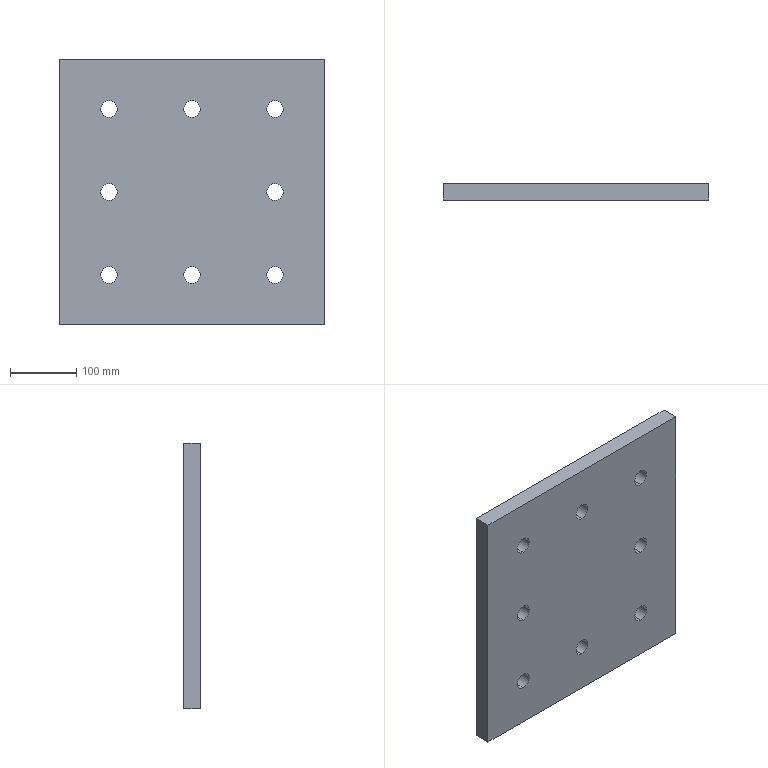Component | SolidWorks | SmallFlange25-2 | 1 solid | 22 faces | box 400 x 25 x 400 mm | volume 3901825 mm3 | cylinder 16 | plane 6 | commonest cylinder face diameters 25 x16 | material Plain Carbon Steel
STEP:
#1=COLOUR_RGB('',0.7922,0.8196,0.9333);
#2=FILL_AREA_STYLE_COLOUR('',#1);
#3=FILL_AREA_STYLE('',(#2));
#4=SURFACE_STYLE_FILL_AREA(#3);
#5=SURFACE_SIDE_STYLE('',(#4));
#6=SURFACE_STYLE_USAGE(.BOTH.,#5);
#7=PRESENTATION_STYLE_ASSIGNMENT((#6));
#8=CARTESIAN_POINT('',(21.257,113.181,151.881));
#9=VERTEX_POINT('',#8);
#10=CARTESIAN_POINT('',(21.257,113.181,152.866));
#11=VERTEX_POINT('',#10);
#12=CARTESIAN_POINT('',(21.257,113.181,152.374));
#13=DIRECTION('',(0.,1.,0.));
#14=DIRECTION('',(0.,0.,1.));
#15=AXIS2_PLACEMENT_3D('',#12,#13,#14);
#16=CIRCLE('',#15,0.4921);
#17=EDGE_CURVE('',#9,#11,#16,.T.);
#18=ORIENTED_EDGE('',*,*,#17,.F.);
#19=CARTESIAN_POINT('',(21.257,114.165,151.881));
#20=VERTEX_POINT('',#19);
#21=CARTESIAN_POINT('',(21.257,113.181,151.881));
#22=DIRECTION('',(0.,1.,0.));
#23=VECTOR('',#22,39.37);
#24=LINE('',#21,#23);
#25=EDGE_CURVE('',#9,#20,#24,.T.);
#26=ORIENTED_EDGE('',*,*,#25,.T.);
#27=CARTESIAN_POINT('',(21.257,114.165,152.866));
#28=VERTEX_POINT('',#27);
#29=CARTESIAN_POINT('',(21.257,114.165,152.374));
#30=DIRECTION('',(0.,1.,0.));
#31=DIRECTION('',(0.,0.,1.));
#32=AXIS2_PLACEMENT_3D('',#29,#30,#31);
#33=CIRCLE('',#32,0.4921);
#34=EDGE_CURVE('',#20,#28,#33,.T.);
#35=ORIENTED_EDGE('',*,*,#34,.T.);
#36=CARTESIAN_POINT('',(21.257,113.181,152.866));
#37=DIRECTION('',(0.,1.,0.));
#38=VECTOR('',#37,39.37);
#39=LINE('',#36,#38);
#40=EDGE_CURVE('',#11,#28,#39,.T.);
#41=ORIENTED_EDGE('',*,*,#40,.F.);
#42=EDGE_LOOP('',(#18,#26,#35,#41));
#43=FACE_OUTER_BOUND('',#42,.T.);
#44=CARTESIAN_POINT('',(21.257,113.181,152.374));
#45=DIRECTION('',(0.,1.,0.));
#46=DIRECTION('',(0.,0.,1.));
#47=AXIS2_PLACEMENT_3D('',#44,#45,#46);
#48=CYLINDRICAL_SURFACE('',#47,0.4921);
#49=ADVANCED_FACE('',(#43),#48,.F.);
#50=CARTESIAN_POINT('',(21.257,113.181,146.96));
#51=VERTEX_POINT('',#50);
#52=CARTESIAN_POINT('',(21.257,113.181,147.944));
#53=VERTEX_POINT('',#52);
#54=CARTESIAN_POINT('',(21.257,113.181,147.452));
#55=DIRECTION('',(0.,1.,0.));
#56=DIRECTION('',(0.,0.,1.));
#57=AXIS2_PLACEMENT_3D('',#54,#55,#56);
#58=CIRCLE('',#57,0.4921);
#59=EDGE_CURVE('',#51,#53,#58,.T.);
#60=ORIENTED_EDGE('',*,*,#59,.F.);
#61=CARTESIAN_POINT('',(21.257,114.165,146.96));
#62=VERTEX_POINT('',#61);
#63=CARTESIAN_POINT('',(21.257,113.181,146.96));
#64=DIRECTION('',(0.,1.,0.));
#65=VECTOR('',#64,39.37);
#66=LINE('',#63,#65);
#67=EDGE_CURVE('',#51,#62,#66,.T.);
#68=ORIENTED_EDGE('',*,*,#67,.T.);
#69=CARTESIAN_POINT('',(21.257,114.165,147.944));
#70=VERTEX_POINT('',#69);
#71=CARTESIAN_POINT('',(21.257,114.165,147.452));
#72=DIRECTION('',(0.,1.,0.));
#73=DIRECTION('',(0.,0.,1.));
#74=AXIS2_PLACEMENT_3D('',#71,#72,#73);
#75=CIRCLE('',#74,0.4921);
#76=EDGE_CURVE('',#62,#70,#75,.T.);
#77=ORIENTED_EDGE('',*,*,#76,.T.);
#78=CARTESIAN_POINT('',(21.257,113.181,147.944));
#79=DIRECTION('',(0.,1.,0.));
#80=VECTOR('',#79,39.37);
#81=LINE('',#78,#80);
#82=EDGE_CURVE('',#53,#70,#81,.T.);
#83=ORIENTED_EDGE('',*,*,#82,.F.);
#84=EDGE_LOOP('',(#60,#68,#77,#83));
#85=FACE_OUTER_BOUND('',#84,.T.);
#86=CARTESIAN_POINT('',(21.257,113.181,147.452));
#87=DIRECTION('',(0.,1.,0.));
#88=DIRECTION('',(0.,0.,1.));
#89=AXIS2_PLACEMENT_3D('',#86,#87,#88);
#90=CYLINDRICAL_SURFACE('',#89,0.4921);
#91=ADVANCED_FACE('',(#85),#90,.F.);
#92=CARTESIAN_POINT('',(31.1,113.181,151.881));
#93=VERTEX_POINT('',#92);
#94=CARTESIAN_POINT('',(31.1,113.181,152.866));
#95=VERTEX_POINT('',#94);
#96=CARTESIAN_POINT('',(31.1,113.181,152.374));
#97=DIRECTION('',(0.,1.,0.));
#98=DIRECTION('',(0.,0.,1.));
#99=AXIS2_PLACEMENT_3D('',#96,#97,#98);
#100=CIRCLE('',#99,0.4921);
#101=EDGE_CURVE('',#93,#95,#100,.T.);
#102=ORIENTED_EDGE('',*,*,#101,.F.);
#103=CARTESIAN_POINT('',(31.1,114.165,151.881));
#104=VERTEX_POINT('',#103);
#105=CARTESIAN_POINT('',(31.1,113.181,151.881));
#106=DIRECTION('',(0.,1.,0.));
#107=VECTOR('',#106,39.37);
#108=LINE('',#105,#107);
#109=EDGE_CURVE('',#93,#104,#108,.T.);
#110=ORIENTED_EDGE('',*,*,#109,.T.);
#111=CARTESIAN_POINT('',(31.1,114.165,152.866));
#112=VERTEX_POINT('',#111);
#113=CARTESIAN_POINT('',(31.1,114.165,152.374));
#114=DIRECTION('',(0.,1.,0.));
#115=DIRECTION('',(0.,0.,1.));
#116=AXIS2_PLACEMENT_3D('',#113,#114,#115);
#117=CIRCLE('',#116,0.4921);
#118=EDGE_CURVE('',#104,#112,#117,.T.);
#119=ORIENTED_EDGE('',*,*,#118,.T.);
#120=CARTESIAN_POINT('',(31.1,113.181,152.866));
#121=DIRECTION('',(0.,1.,0.));
#122=VECTOR('',#121,39.37);
#123=LINE('',#120,#122);
#124=EDGE_CURVE('',#95,#112,#123,.T.);
#125=ORIENTED_EDGE('',*,*,#124,.F.);
#126=EDGE_LOOP('',(#102,#110,#119,#125));
#127=FACE_OUTER_BOUND('',#126,.T.);
#128=CARTESIAN_POINT('',(31.1,113.181,152.374));
#129=DIRECTION('',(0.,1.,0.));
#130=DIRECTION('',(0.,0.,1.));
#131=AXIS2_PLACEMENT_3D('',#128,#129,#130);
#132=CYLINDRICAL_SURFACE('',#131,0.4921);
#133=ADVANCED_FACE('',(#127),#132,.F.);
#134=CARTESIAN_POINT('',(26.179,113.181,151.881));
#135=VERTEX_POINT('',#134);
#136=CARTESIAN_POINT('',(26.179,113.181,152.866));
#137=VERTEX_POINT('',#136);
#138=CARTESIAN_POINT('',(26.179,113.181,152.374));
#139=DIRECTION('',(0.,1.,0.));
#140=DIRECTION('',(0.,0.,1.));
#141=AXIS2_PLACEMENT_3D('',#138,#139,#140);
#142=CIRCLE('',#141,0.4921);
#143=EDGE_CURVE('',#135,#137,#142,.T.);
#144=ORIENTED_EDGE('',*,*,#143,.F.);
#145=CARTESIAN_POINT('',(26.179,114.165,151.881));
#146=VERTEX_POINT('',#145);
#147=CARTESIAN_POINT('',(26.179,113.181,151.881));
#148=DIRECTION('',(0.,1.,0.));
#149=VECTOR('',#148,39.37);
#150=LINE('',#147,#149);
#151=EDGE_CURVE('',#135,#146,#150,.T.);
#152=ORIENTED_EDGE('',*,*,#151,.T.);
#153=CARTESIAN_POINT('',(26.179,114.165,152.866));
#154=VERTEX_POINT('',#153);
#155=CARTESIAN_POINT('',(26.179,114.165,152.374));
#156=DIRECTION('',(0.,1.,0.));
#157=DIRECTION('',(0.,0.,1.));
#158=AXIS2_PLACEMENT_3D('',#155,#156,#157);
#159=CIRCLE('',#158,0.4921);
#160=EDGE_CURVE('',#146,#154,#159,.T.);
#161=ORIENTED_EDGE('',*,*,#160,.T.);
#162=CARTESIAN_POINT('',(26.179,113.181,152.866));
#163=DIRECTION('',(0.,1.,0.));
#164=VECTOR('',#163,39.37);
#165=LINE('',#162,#164);
#166=EDGE_CURVE('',#137,#154,#165,.T.);
#167=ORIENTED_EDGE('',*,*,#166,.F.);
#168=EDGE_LOOP('',(#144,#152,#161,#167));
#169=FACE_OUTER_BOUND('',#168,.T.);
#170=CARTESIAN_POINT('',(26.179,113.181,152.374));
#171=DIRECTION('',(0.,1.,0.));
#172=DIRECTION('',(0.,0.,1.));
#173=AXIS2_PLACEMENT_3D('',#170,#171,#172);
#174=CYLINDRICAL_SURFACE('',#173,0.4921);
#175=ADVANCED_FACE('',(#169),#174,.F.);
#176=CARTESIAN_POINT('',(31.1,113.181,146.96));
#177=VERTEX_POINT('',#176);
#178=CARTESIAN_POINT('',(31.1,113.181,147.944));
#179=VERTEX_POINT('',#178);
#180=CARTESIAN_POINT('',(31.1,113.181,147.452));
#181=DIRECTION('',(0.,1.,0.));
#182=DIRECTION('',(0.,0.,1.));
#183=AXIS2_PLACEMENT_3D('',#180,#181,#182);
#184=CIRCLE('',#183,0.4921);
#185=EDGE_CURVE('',#177,#179,#184,.T.);
#186=ORIENTED_EDGE('',*,*,#185,.F.);
#187=CARTESIAN_POINT('',(31.1,114.165,146.96));
#188=VERTEX_POINT('',#187);
#189=CARTESIAN_POINT('',(31.1,113.181,146.96));
#190=DIRECTION('',(0.,1.,0.));
#191=VECTOR('',#190,39.37);
#192=LINE('',#189,#191);
#193=EDGE_CURVE('',#177,#188,#192,.T.);
#194=ORIENTED_EDGE('',*,*,#193,.T.);
#195=CARTESIAN_POINT('',(31.1,114.165,147.944));
#196=VERTEX_POINT('',#195);
#197=CARTESIAN_POINT('',(31.1,114.165,147.452));
#198=DIRECTION('',(0.,1.,0.));
#199=DIRECTION('',(0.,0.,1.));
#200=AXIS2_PLACEMENT_3D('',#197,#198,#199);
#201=CIRCLE('',#200,0.4921);
#202=EDGE_CURVE('',#188,#196,#201,.T.);
#203=ORIENTED_EDGE('',*,*,#202,.T.);
#204=CARTESIAN_POINT('',(31.1,113.181,147.944));
#205=DIRECTION('',(0.,1.,0.));
#206=VECTOR('',#205,39.37);
#207=LINE('',#204,#206);
#208=EDGE_CURVE('',#179,#196,#207,.T.);
#209=ORIENTED_EDGE('',*,*,#208,.F.);
#210=EDGE_LOOP('',(#186,#194,#203,#209));
#211=FACE_OUTER_BOUND('',#210,.T.);
#212=CARTESIAN_POINT('',(31.1,113.181,147.452));
#213=DIRECTION('',(0.,1.,0.));
#214=DIRECTION('',(0.,0.,1.));
#215=AXIS2_PLACEMENT_3D('',#212,#213,#214);
#216=CYLINDRICAL_SURFACE('',#215,0.4921);
#217=ADVANCED_FACE('',(#211),#216,.F.);
#218=CARTESIAN_POINT('',(31.1,113.181,142.039));
#219=VERTEX_POINT('',#218);
#220=CARTESIAN_POINT('',(31.1,113.181,143.023));
#221=VERTEX_POINT('',#220);
#222=CARTESIAN_POINT('',(31.1,113.181,142.531));
#223=DIRECTION('',(0.,1.,0.));
#224=DIRECTION('',(0.,0.,1.));
#225=AXIS2_PLACEMENT_3D('',#222,#223,#224);
#226=CIRCLE('',#225,0.4921);
#227=EDGE_CURVE('',#219,#221,#226,.T.);
#228=ORIENTED_EDGE('',*,*,#227,.F.);
#229=CARTESIAN_POINT('',(31.1,114.165,142.039));
#230=VERTEX_POINT('',#229);
#231=CARTESIAN_POINT('',(31.1,113.181,142.039));
#232=DIRECTION('',(0.,1.,0.));
#233=VECTOR('',#232,39.37);
#234=LINE('',#231,#233);
#235=EDGE_CURVE('',#219,#230,#234,.T.);
#236=ORIENTED_EDGE('',*,*,#235,.T.);
#237=CARTESIAN_POINT('',(31.1,114.165,143.023));
#238=VERTEX_POINT('',#237);
#239=CARTESIAN_POINT('',(31.1,114.165,142.531));
#240=DIRECTION('',(0.,1.,0.));
#241=DIRECTION('',(0.,0.,1.));
#242=AXIS2_PLACEMENT_3D('',#239,#240,#241);
#243=CIRCLE('',#242,0.4921);
#244=EDGE_CURVE('',#230,#238,#243,.T.);
#245=ORIENTED_EDGE('',*,*,#244,.T.);
#246=CARTESIAN_POINT('',(31.1,113.181,143.023));
#247=DIRECTION('',(0.,1.,0.));
#248=VECTOR('',#247,39.37);
#249=LINE('',#246,#248);
#250=EDGE_CURVE('',#221,#238,#249,.T.);
#251=ORIENTED_EDGE('',*,*,#250,.F.);
#252=EDGE_LOOP('',(#228,#236,#245,#251));
#253=FACE_OUTER_BOUND('',#252,.T.);
#254=CARTESIAN_POINT('',(31.1,113.181,142.531));
#255=DIRECTION('',(0.,1.,0.));
#256=DIRECTION('',(0.,0.,1.));
#257=AXIS2_PLACEMENT_3D('',#254,#255,#256);
#258=CYLINDRICAL_SURFACE('',#257,0.4921);
#259=ADVANCED_FACE('',(#253),#258,.F.);
#260=CARTESIAN_POINT('',(26.179,113.181,142.039));
#261=VERTEX_POINT('',#260);
#262=CARTESIAN_POINT('',(26.179,113.181,143.023));
#263=VERTEX_POINT('',#262);
#264=CARTESIAN_POINT('',(26.179,113.181,142.531));
#265=DIRECTION('',(0.,1.,0.));
#266=DIRECTION('',(0.,0.,1.));
#267=AXIS2_PLACEMENT_3D('',#264,#265,#266);
#268=CIRCLE('',#267,0.4921);
#269=EDGE_CURVE('',#261,#263,#268,.T.);
#270=ORIENTED_EDGE('',*,*,#269,.F.);
#271=CARTESIAN_POINT('',(26.179,114.165,142.039));
#272=VERTEX_POINT('',#271);
#273=CARTESIAN_POINT('',(26.179,113.181,142.039));
#274=DIRECTION('',(0.,1.,0.));
#275=VECTOR('',#274,39.37);
#276=LINE('',#273,#275);
#277=EDGE_CURVE('',#261,#272,#276,.T.);
#278=ORIENTED_EDGE('',*,*,#277,.T.);
#279=CARTESIAN_POINT('',(26.179,114.165,143.023));
#280=VERTEX_POINT('',#279);
#281=CARTESIAN_POINT('',(26.179,114.165,142.531));
#282=DIRECTION('',(0.,1.,0.));
#283=DIRECTION('',(0.,0.,1.));
#284=AXIS2_PLACEMENT_3D('',#281,#282,#283);
#285=CIRCLE('',#284,0.4921);
#286=EDGE_CURVE('',#272,#280,#285,.T.);
#287=ORIENTED_EDGE('',*,*,#286,.T.);
#288=CARTESIAN_POINT('',(26.179,113.181,143.023));
#289=DIRECTION('',(0.,1.,0.));
#290=VECTOR('',#289,39.37);
#291=LINE('',#288,#290);
#292=EDGE_CURVE('',#263,#280,#291,.T.);
#293=ORIENTED_EDGE('',*,*,#292,.F.);
#294=EDGE_LOOP('',(#270,#278,#287,#293));
#295=FACE_OUTER_BOUND('',#294,.T.);
#296=CARTESIAN_POINT('',(26.179,113.181,142.531));
#297=DIRECTION('',(0.,1.,0.));
#298=DIRECTION('',(0.,0.,1.));
#299=AXIS2_PLACEMENT_3D('',#296,#297,#298);
#300=CYLINDRICAL_SURFACE('',#299,0.4921);
#301=ADVANCED_FACE('',(#295),#300,.F.);
#302=CARTESIAN_POINT('',(21.257,113.181,142.039));
#303=VERTEX_POINT('',#302);
#304=CARTESIAN_POINT('',(21.257,113.181,143.023));
#305=VERTEX_POINT('',#304);
#306=CARTESIAN_POINT('',(21.257,113.181,142.531));
#307=DIRECTION('',(0.,1.,0.));
#308=DIRECTION('',(0.,0.,1.));
#309=AXIS2_PLACEMENT_3D('',#306,#307,#308);
#310=CIRCLE('',#309,0.4921);
#311=EDGE_CURVE('',#303,#305,#310,.T.);
#312=ORIENTED_EDGE('',*,*,#311,.F.);
#313=CARTESIAN_POINT('',(21.257,114.165,142.039));
#314=VERTEX_POINT('',#313);
#315=CARTESIAN_POINT('',(21.257,113.181,142.039));
#316=DIRECTION('',(0.,1.,0.));
#317=VECTOR('',#316,39.37);
#318=LINE('',#315,#317);
#319=EDGE_CURVE('',#303,#314,#318,.T.);
#320=ORIENTED_EDGE('',*,*,#319,.T.);
#321=CARTESIAN_POINT('',(21.257,114.165,143.023));
#322=VERTEX_POINT('',#321);
#323=CARTESIAN_POINT('',(21.257,114.165,142.531));
#324=DIRECTION('',(0.,1.,0.));
#325=DIRECTION('',(0.,0.,1.));
#326=AXIS2_PLACEMENT_3D('',#323,#324,#325);
#327=CIRCLE('',#326,0.4921);
#328=EDGE_CURVE('',#314,#322,#327,.T.);
#329=ORIENTED_EDGE('',*,*,#328,.T.);
#330=CARTESIAN_POINT('',(21.257,113.181,143.023));
#331=DIRECTION('',(0.,1.,0.));
#332=VECTOR('',#331,39.37);
#333=LINE('',#330,#332);
#334=EDGE_CURVE('',#305,#322,#333,.T.);
#335=ORIENTED_EDGE('',*,*,#334,.F.);
#336=EDGE_LOOP('',(#312,#320,#329,#335));
#337=FACE_OUTER_BOUND('',#336,.T.);
#338=CARTESIAN_POINT('',(21.257,113.181,142.531));
#339=DIRECTION('',(0.,1.,0.));
#340=DIRECTION('',(0.,0.,1.));
#341=AXIS2_PLACEMENT_3D('',#338,#339,#340);
#342=CYLINDRICAL_SURFACE('',#341,0.4921);
#343=ADVANCED_FACE('',(#337),#342,.F.);
#344=CARTESIAN_POINT('',(34.053,114.165,155.326));
#345=VERTEX_POINT('',#344);
#346=CARTESIAN_POINT('',(34.053,114.165,139.578));
#347=VERTEX_POINT('',#346);
#348=CARTESIAN_POINT('',(34.053,114.165,139.578));
#349=DIRECTION('',(-0.,0.,-1.));
#350=VECTOR('',#349,39.37);
#351=LINE('',#348,#350);
#352=EDGE_CURVE('',#345,#347,#351,.T.);
#353=ORIENTED_EDGE('',*,*,#352,.F.);
#354=CARTESIAN_POINT('',(34.053,113.181,155.326));
#355=VERTEX_POINT('',#354);
#356=CARTESIAN_POINT('',(34.053,113.181,155.326));
#357=DIRECTION('',(0.,1.,0.));
#358=VECTOR('',#357,39.37);
#359=LINE('',#356,#358);
#360=EDGE_CURVE('',#355,#345,#359,.T.);
#361=ORIENTED_EDGE('',*,*,#360,.F.);
#362=CARTESIAN_POINT('',(34.053,113.181,139.578));
#363=VERTEX_POINT('',#362);
#364=CARTESIAN_POINT('',(34.053,113.181,139.578));
#365=DIRECTION('',(-0.,0.,-1.));
#366=VECTOR('',#365,39.37);
#367=LINE('',#364,#366);
#368=EDGE_CURVE('',#355,#363,#367,.T.);
#369=ORIENTED_EDGE('',*,*,#368,.T.);
#370=CARTESIAN_POINT('',(34.053,113.181,139.578));
#371=DIRECTION('',(0.,1.,0.));
#372=VECTOR('',#371,39.37);
#373=LINE('',#370,#372);
#374=EDGE_CURVE('',#363,#347,#373,.T.);
#375=ORIENTED_EDGE('',*,*,#374,.T.);
#376=EDGE_LOOP('',(#353,#361,#369,#375));
#377=FACE_OUTER_BOUND('',#376,.T.);
#378=CARTESIAN_POINT('',(34.053,113.181,139.578));
#379=DIRECTION('',(1.,0.,-0.));
#380=DIRECTION('',(-0.,0.,-1.));
#381=AXIS2_PLACEMENT_3D('',#378,#379,#380);
#382=PLANE('',#381);
#383=ADVANCED_FACE('',(#377),#382,.T.);
#384=CARTESIAN_POINT('',(18.305,114.165,155.326));
#385=VERTEX_POINT('',#384);
#386=CARTESIAN_POINT('',(18.305,114.165,155.326));
#387=DIRECTION('',(1.,0.,0.));
#388=VECTOR('',#387,39.37);
#389=LINE('',#386,#388);
#390=EDGE_CURVE('',#385,#345,#389,.T.);
#391=ORIENTED_EDGE('',*,*,#390,.F.);
#392=CARTESIAN_POINT('',(18.305,113.181,155.326));
#393=VERTEX_POINT('',#392);
#394=CARTESIAN_POINT('',(18.305,113.181,155.326));
#395=DIRECTION('',(0.,1.,0.));
#396=VECTOR('',#395,39.37);
#397=LINE('',#394,#396);
#398=EDGE_CURVE('',#393,#385,#397,.T.);
#399=ORIENTED_EDGE('',*,*,#398,.F.);
#400=CARTESIAN_POINT('',(18.305,113.181,155.326));
#401=DIRECTION('',(1.,0.,0.));
#402=VECTOR('',#401,39.37);
#403=LINE('',#400,#402);
#404=EDGE_CURVE('',#393,#355,#403,.T.);
#405=ORIENTED_EDGE('',*,*,#404,.T.);
#406=ORIENTED_EDGE('',*,*,#360,.T.);
#407=EDGE_LOOP('',(#391,#399,#405,#406));
#408=FACE_OUTER_BOUND('',#407,.T.);
#409=CARTESIAN_POINT('',(18.305,113.181,155.326));
#410=DIRECTION('',(0.,0.,1.));
#411=DIRECTION('',(1.,0.,0.));
#412=AXIS2_PLACEMENT_3D('',#409,#410,#411);
#413=PLANE('',#412);
#414=ADVANCED_FACE('',(#408),#413,.T.);
#415=CARTESIAN_POINT('',(18.305,114.165,139.578));
#416=VERTEX_POINT('',#415);
#417=CARTESIAN_POINT('',(18.305,114.165,139.578));
#418=DIRECTION('',(0.,0.,1.));
#419=VECTOR('',#418,39.37);
#420=LINE('',#417,#419);
#421=EDGE_CURVE('',#416,#385,#420,.T.);
#422=ORIENTED_EDGE('',*,*,#421,.F.);
#423=CARTESIAN_POINT('',(18.305,113.181,139.578));
#424=VERTEX_POINT('',#423);
#425=CARTESIAN_POINT('',(18.305,113.181,139.578));
#426=DIRECTION('',(0.,1.,0.));
#427=VECTOR('',#426,39.37);
#428=LINE('',#425,#427);
#429=EDGE_CURVE('',#424,#416,#428,.T.);
#430=ORIENTED_EDGE('',*,*,#429,.F.);
#431=CARTESIAN_POINT('',(18.305,113.181,139.578));
#432=DIRECTION('',(0.,0.,1.));
#433=VECTOR('',#432,39.37);
#434=LINE('',#431,#433);
#435=EDGE_CURVE('',#424,#393,#434,.T.);
#436=ORIENTED_EDGE('',*,*,#435,.T.);
#437=ORIENTED_EDGE('',*,*,#398,.T.);
#438=EDGE_LOOP('',(#422,#430,#436,#437));
#439=FACE_OUTER_BOUND('',#438,.T.);
#440=CARTESIAN_POINT('',(18.305,113.181,139.578));
#441=DIRECTION('',(-1.,0.,0.));
#442=DIRECTION('',(0.,0.,1.));
#443=AXIS2_PLACEMENT_3D('',#440,#441,#442);
#444=PLANE('',#443);
#445=ADVANCED_FACE('',(#439),#444,.T.);
#446=CARTESIAN_POINT('',(18.305,114.165,139.578));
#447=DIRECTION('',(-1.,0.,0.));
#448=VECTOR('',#447,39.37);
#449=LINE('',#446,#448);
#450=EDGE_CURVE('',#347,#416,#449,.T.);
#451=ORIENTED_EDGE('',*,*,#450,.F.);
#452=ORIENTED_EDGE('',*,*,#374,.F.);
#453=CARTESIAN_POINT('',(18.305,113.181,139.578));
#454=DIRECTION('',(-1.,0.,0.));
#455=VECTOR('',#454,39.37);
#456=LINE('',#453,#455);
#457=EDGE_CURVE('',#363,#424,#456,.T.);
#458=ORIENTED_EDGE('',*,*,#457,.T.);
#459=ORIENTED_EDGE('',*,*,#429,.T.);
#460=EDGE_LOOP('',(#451,#452,#458,#459));
#461=FACE_OUTER_BOUND('',#460,.T.);
#462=CARTESIAN_POINT('',(18.305,113.181,139.578));
#463=DIRECTION('',(0.,0.,-1.));
#464=DIRECTION('',(-1.,0.,0.));
#465=AXIS2_PLACEMENT_3D('',#462,#463,#464);
#466=PLANE('',#465);
#467=ADVANCED_FACE('',(#461),#466,.T.);
#468=CARTESIAN_POINT('',(21.257,113.181,152.374));
#469=DIRECTION('',(0.,1.,0.));
#470=DIRECTION('',(0.,0.,1.));
#471=AXIS2_PLACEMENT_3D('',#468,#469,#470);
#472=CIRCLE('',#471,0.4921);
#473=EDGE_CURVE('',#11,#9,#472,.T.);
#474=ORIENTED_EDGE('',*,*,#473,.T.);
#475=ORIENTED_EDGE('',*,*,#17,.T.);
#476=EDGE_LOOP('',(#474,#475));
#477=FACE_BOUND('',#476,.T.);
#478=CARTESIAN_POINT('',(21.257,113.181,147.452));
#479=DIRECTION('',(0.,1.,0.));
#480=DIRECTION('',(0.,0.,1.));
#481=AXIS2_PLACEMENT_3D('',#478,#479,#480);
#482=CIRCLE('',#481,0.4921);
#483=EDGE_CURVE('',#53,#51,#482,.T.);
#484=ORIENTED_EDGE('',*,*,#483,.T.);
#485=ORIENTED_EDGE('',*,*,#59,.T.);
#486=EDGE_LOOP('',(#484,#485));
#487=FACE_BOUND('',#486,.T.);
#488=CARTESIAN_POINT('',(31.1,113.181,152.374));
#489=DIRECTION('',(0.,1.,0.));
#490=DIRECTION('',(0.,0.,1.));
#491=AXIS2_PLACEMENT_3D('',#488,#489,#490);
#492=CIRCLE('',#491,0.4921);
#493=EDGE_CURVE('',#95,#93,#492,.T.);
#494=ORIENTED_EDGE('',*,*,#493,.T.);
#495=ORIENTED_EDGE('',*,*,#101,.T.);
#496=EDGE_LOOP('',(#494,#495));
#497=FACE_BOUND('',#496,.T.);
#498=CARTESIAN_POINT('',(26.179,113.181,152.374));
#499=DIRECTION('',(0.,1.,0.));
#500=DIRECTION('',(0.,0.,1.));
#501=AXIS2_PLACEMENT_3D('',#498,#499,#500);
#502=CIRCLE('',#501,0.4921);
#503=EDGE_CURVE('',#137,#135,#502,.T.);
#504=ORIENTED_EDGE('',*,*,#503,.T.);
#505=ORIENTED_EDGE('',*,*,#143,.T.);
#506=EDGE_LOOP('',(#504,#505));
#507=FACE_BOUND('',#506,.T.);
#508=CARTESIAN_POINT('',(31.1,113.181,147.452));
#509=DIRECTION('',(0.,1.,0.));
#510=DIRECTION('',(0.,0.,1.));
#511=AXIS2_PLACEMENT_3D('',#508,#509,#510);
#512=CIRCLE('',#511,0.4921);
#513=EDGE_CURVE('',#179,#177,#512,.T.);
#514=ORIENTED_EDGE('',*,*,#513,.T.);
#515=ORIENTED_EDGE('',*,*,#185,.T.);
#516=EDGE_LOOP('',(#514,#515));
#517=FACE_BOUND('',#516,.T.);
#518=CARTESIAN_POINT('',(31.1,113.181,142.531));
#519=DIRECTION('',(0.,1.,0.));
#520=DIRECTION('',(0.,0.,1.));
#521=AXIS2_PLACEMENT_3D('',#518,#519,#520);
#522=CIRCLE('',#521,0.4921);
#523=EDGE_CURVE('',#221,#219,#522,.T.);
#524=ORIENTED_EDGE('',*,*,#523,.T.);
#525=ORIENTED_EDGE('',*,*,#227,.T.);
#526=EDGE_LOOP('',(#524,#525));
#527=FACE_BOUND('',#526,.T.);
#528=CARTESIAN_POINT('',(26.179,113.181,142.531));
#529=DIRECTION('',(0.,1.,0.));
#530=DIRECTION('',(0.,0.,1.));
#531=AXIS2_PLACEMENT_3D('',#528,#529,#530);
#532=CIRCLE('',#531,0.4921);
#533=EDGE_CURVE('',#263,#261,#532,.T.);
#534=ORIENTED_EDGE('',*,*,#533,.T.);
#535=ORIENTED_EDGE('',*,*,#269,.T.);
#536=EDGE_LOOP('',(#534,#535));
#537=FACE_BOUND('',#536,.T.);
#538=CARTESIAN_POINT('',(21.257,113.181,142.531));
#539=DIRECTION('',(0.,1.,0.));
#540=DIRECTION('',(0.,0.,1.));
#541=AXIS2_PLACEMENT_3D('',#538,#539,#540);
#542=CIRCLE('',#541,0.4921);
#543=EDGE_CURVE('',#305,#303,#542,.T.);
#544=ORIENTED_EDGE('',*,*,#543,.T.);
#545=ORIENTED_EDGE('',*,*,#311,.T.);
#546=EDGE_LOOP('',(#544,#545));
#547=FACE_BOUND('',#546,.T.);
#548=ORIENTED_EDGE('',*,*,#368,.F.);
#549=ORIENTED_EDGE('',*,*,#404,.F.);
#550=ORIENTED_EDGE('',*,*,#435,.F.);
#551=ORIENTED_EDGE('',*,*,#457,.F.);
#552=EDGE_LOOP('',(#548,#549,#550,#551));
#553=FACE_OUTER_BOUND('',#552,.T.);
#554=CARTESIAN_POINT('',(26.179,113.181,147.452));
#555=DIRECTION('',(0.,1.,0.));
#556=DIRECTION('',(0.,0.,1.));
#557=AXIS2_PLACEMENT_3D('',#554,#555,#556);
#558=PLANE('',#557);
#559=ADVANCED_FACE('',(#477,#487,#497,#507,#517,#527,#537,#547,#553),#558,.F.);
#560=CARTESIAN_POINT('',(21.257,114.165,152.374));
#561=DIRECTION('',(0.,1.,0.));
#562=DIRECTION('',(0.,0.,1.));
#563=AXIS2_PLACEMENT_3D('',#560,#561,#562);
#564=CIRCLE('',#563,0.4921);
#565=EDGE_CURVE('',#28,#20,#564,.T.);
#566=ORIENTED_EDGE('',*,*,#565,.F.);
#567=ORIENTED_EDGE('',*,*,#34,.F.);
#568=EDGE_LOOP('',(#566,#567));
#569=FACE_BOUND('',#568,.T.);
#570=CARTESIAN_POINT('',(21.257,114.165,147.452));
#571=DIRECTION('',(0.,1.,0.));
#572=DIRECTION('',(0.,0.,1.));
#573=AXIS2_PLACEMENT_3D('',#570,#571,#572);
#574=CIRCLE('',#573,0.4921);
#575=EDGE_CURVE('',#70,#62,#574,.T.);
#576=ORIENTED_EDGE('',*,*,#575,.F.);
#577=ORIENTED_EDGE('',*,*,#76,.F.);
#578=EDGE_LOOP('',(#576,#577));
#579=FACE_BOUND('',#578,.T.);
#580=CARTESIAN_POINT('',(31.1,114.165,152.374));
#581=DIRECTION('',(0.,1.,0.));
#582=DIRECTION('',(0.,0.,1.));
#583=AXIS2_PLACEMENT_3D('',#580,#581,#582);
#584=CIRCLE('',#583,0.4921);
#585=EDGE_CURVE('',#112,#104,#584,.T.);
#586=ORIENTED_EDGE('',*,*,#585,.F.);
#587=ORIENTED_EDGE('',*,*,#118,.F.);
#588=EDGE_LOOP('',(#586,#587));
#589=FACE_BOUND('',#588,.T.);
#590=CARTESIAN_POINT('',(26.179,114.165,152.374));
#591=DIRECTION('',(0.,1.,0.));
#592=DIRECTION('',(0.,0.,1.));
#593=AXIS2_PLACEMENT_3D('',#590,#591,#592);
#594=CIRCLE('',#593,0.4921);
#595=EDGE_CURVE('',#154,#146,#594,.T.);
#596=ORIENTED_EDGE('',*,*,#595,.F.);
#597=ORIENTED_EDGE('',*,*,#160,.F.);
#598=EDGE_LOOP('',(#596,#597));
#599=FACE_BOUND('',#598,.T.);
#600=CARTESIAN_POINT('',(31.1,114.165,147.452));
#601=DIRECTION('',(0.,1.,0.));
#602=DIRECTION('',(0.,0.,1.));
#603=AXIS2_PLACEMENT_3D('',#600,#601,#602);
#604=CIRCLE('',#603,0.4921);
#605=EDGE_CURVE('',#196,#188,#604,.T.);
#606=ORIENTED_EDGE('',*,*,#605,.F.);
#607=ORIENTED_EDGE('',*,*,#202,.F.);
#608=EDGE_LOOP('',(#606,#607));
#609=FACE_BOUND('',#608,.T.);
#610=CARTESIAN_POINT('',(31.1,114.165,142.531));
#611=DIRECTION('',(0.,1.,0.));
#612=DIRECTION('',(0.,0.,1.));
#613=AXIS2_PLACEMENT_3D('',#610,#611,#612);
#614=CIRCLE('',#613,0.4921);
#615=EDGE_CURVE('',#238,#230,#614,.T.);
#616=ORIENTED_EDGE('',*,*,#615,.F.);
#617=ORIENTED_EDGE('',*,*,#244,.F.);
#618=EDGE_LOOP('',(#616,#617));
#619=FACE_BOUND('',#618,.T.);
#620=CARTESIAN_POINT('',(26.179,114.165,142.531));
#621=DIRECTION('',(0.,1.,0.));
#622=DIRECTION('',(0.,0.,1.));
#623=AXIS2_PLACEMENT_3D('',#620,#621,#622);
#624=CIRCLE('',#623,0.4921);
#625=EDGE_CURVE('',#280,#272,#624,.T.);
#626=ORIENTED_EDGE('',*,*,#625,.F.);
#627=ORIENTED_EDGE('',*,*,#286,.F.);
#628=EDGE_LOOP('',(#626,#627));
#629=FACE_BOUND('',#628,.T.);
#630=CARTESIAN_POINT('',(21.257,114.165,142.531));
#631=DIRECTION('',(0.,1.,0.));
#632=DIRECTION('',(0.,0.,1.));
#633=AXIS2_PLACEMENT_3D('',#630,#631,#632);
#634=CIRCLE('',#633,0.4921);
#635=EDGE_CURVE('',#322,#314,#634,.T.);
#636=ORIENTED_EDGE('',*,*,#635,.F.);
#637=ORIENTED_EDGE('',*,*,#328,.F.);
#638=EDGE_LOOP('',(#636,#637));
#639=FACE_BOUND('',#638,.T.);
#640=ORIENTED_EDGE('',*,*,#352,.T.);
#641=ORIENTED_EDGE('',*,*,#450,.T.);
#642=ORIENTED_EDGE('',*,*,#421,.T.);
#643=ORIENTED_EDGE('',*,*,#390,.T.);
#644=EDGE_LOOP('',(#640,#641,#642,#643));
#645=FACE_OUTER_BOUND('',#644,.T.);
#646=CARTESIAN_POINT('',(26.179,114.165,147.452));
#647=DIRECTION('',(0.,1.,0.));
#648=DIRECTION('',(0.,0.,1.));
#649=AXIS2_PLACEMENT_3D('',#646,#647,#648);
#650=PLANE('',#649);
#651=ADVANCED_FACE('',(#569,#579,#589,#599,#609,#619,#629,#639,#645),#650,.T.);
#652=ORIENTED_EDGE('',*,*,#319,.F.);
#653=ORIENTED_EDGE('',*,*,#543,.F.);
#654=ORIENTED_EDGE('',*,*,#334,.T.);
#655=ORIENTED_EDGE('',*,*,#635,.T.);
#656=EDGE_LOOP('',(#652,#653,#654,#655));
#657=FACE_OUTER_BOUND('',#656,.T.);
#658=CARTESIAN_POINT('',(21.257,113.181,142.531));
#659=DIRECTION('',(0.,1.,0.));
#660=DIRECTION('',(0.,0.,1.));
#661=AXIS2_PLACEMENT_3D('',#658,#659,#660);
#662=CYLINDRICAL_SURFACE('',#661,0.4921);
#663=ADVANCED_FACE('',(#657),#662,.F.);
#664=ORIENTED_EDGE('',*,*,#277,.F.);
#665=ORIENTED_EDGE('',*,*,#533,.F.);
#666=ORIENTED_EDGE('',*,*,#292,.T.);
#667=ORIENTED_EDGE('',*,*,#625,.T.);
#668=EDGE_LOOP('',(#664,#665,#666,#667));
#669=FACE_OUTER_BOUND('',#668,.T.);
#670=CARTESIAN_POINT('',(26.179,113.181,142.531));
#671=DIRECTION('',(0.,1.,0.));
#672=DIRECTION('',(0.,0.,1.));
#673=AXIS2_PLACEMENT_3D('',#670,#671,#672);
#674=CYLINDRICAL_SURFACE('',#673,0.4921);
#675=ADVANCED_FACE('',(#669),#674,.F.);
#676=ORIENTED_EDGE('',*,*,#235,.F.);
#677=ORIENTED_EDGE('',*,*,#523,.F.);
#678=ORIENTED_EDGE('',*,*,#250,.T.);
#679=ORIENTED_EDGE('',*,*,#615,.T.);
#680=EDGE_LOOP('',(#676,#677,#678,#679));
#681=FACE_OUTER_BOUND('',#680,.T.);
#682=CARTESIAN_POINT('',(31.1,113.181,142.531));
#683=DIRECTION('',(0.,1.,0.));
#684=DIRECTION('',(0.,0.,1.));
#685=AXIS2_PLACEMENT_3D('',#682,#683,#684);
#686=CYLINDRICAL_SURFACE('',#685,0.4921);
#687=ADVANCED_FACE('',(#681),#686,.F.);
#688=ORIENTED_EDGE('',*,*,#193,.F.);
#689=ORIENTED_EDGE('',*,*,#513,.F.);
#690=ORIENTED_EDGE('',*,*,#208,.T.);
#691=ORIENTED_EDGE('',*,*,#605,.T.);
#692=EDGE_LOOP('',(#688,#689,#690,#691));
#693=FACE_OUTER_BOUND('',#692,.T.);
#694=CARTESIAN_POINT('',(31.1,113.181,147.452));
#695=DIRECTION('',(0.,1.,0.));
#696=DIRECTION('',(0.,0.,1.));
#697=AXIS2_PLACEMENT_3D('',#694,#695,#696);
#698=CYLINDRICAL_SURFACE('',#697,0.4921);
#699=ADVANCED_FACE('',(#693),#698,.F.);
#700=ORIENTED_EDGE('',*,*,#151,.F.);
#701=ORIENTED_EDGE('',*,*,#503,.F.);
#702=ORIENTED_EDGE('',*,*,#166,.T.);
#703=ORIENTED_EDGE('',*,*,#595,.T.);
#704=EDGE_LOOP('',(#700,#701,#702,#703));
#705=FACE_OUTER_BOUND('',#704,.T.);
#706=CARTESIAN_POINT('',(26.179,113.181,152.374));
#707=DIRECTION('',(0.,1.,0.));
#708=DIRECTION('',(0.,0.,1.));
#709=AXIS2_PLACEMENT_3D('',#706,#707,#708);
#710=CYLINDRICAL_SURFACE('',#709,0.4921);
#711=ADVANCED_FACE('',(#705),#710,.F.);
#712=ORIENTED_EDGE('',*,*,#109,.F.);
#713=ORIENTED_EDGE('',*,*,#493,.F.);
#714=ORIENTED_EDGE('',*,*,#124,.T.);
#715=ORIENTED_EDGE('',*,*,#585,.T.);
#716=EDGE_LOOP('',(#712,#713,#714,#715));
#717=FACE_OUTER_BOUND('',#716,.T.);
#718=CARTESIAN_POINT('',(31.1,113.181,152.374));
#719=DIRECTION('',(0.,1.,0.));
#720=DIRECTION('',(0.,0.,1.));
#721=AXIS2_PLACEMENT_3D('',#718,#719,#720);
#722=CYLINDRICAL_SURFACE('',#721,0.4921);
#723=ADVANCED_FACE('',(#717),#722,.F.);
#724=ORIENTED_EDGE('',*,*,#67,.F.);
#725=ORIENTED_EDGE('',*,*,#483,.F.);
#726=ORIENTED_EDGE('',*,*,#82,.T.);
#727=ORIENTED_EDGE('',*,*,#575,.T.);
#728=EDGE_LOOP('',(#724,#725,#726,#727));
#729=FACE_OUTER_BOUND('',#728,.T.);
#730=CARTESIAN_POINT('',(21.257,113.181,147.452));
#731=DIRECTION('',(0.,1.,0.));
#732=DIRECTION('',(0.,0.,1.));
#733=AXIS2_PLACEMENT_3D('',#730,#731,#732);
#734=CYLINDRICAL_SURFACE('',#733,0.4921);
#735=ADVANCED_FACE('',(#729),#734,.F.);
#736=ORIENTED_EDGE('',*,*,#25,.F.);
#737=ORIENTED_EDGE('',*,*,#473,.F.);
#738=ORIENTED_EDGE('',*,*,#40,.T.);
#739=ORIENTED_EDGE('',*,*,#565,.T.);
#740=EDGE_LOOP('',(#736,#737,#738,#739));
#741=FACE_OUTER_BOUND('',#740,.T.);
#742=CARTESIAN_POINT('',(21.257,113.181,152.374));
#743=DIRECTION('',(0.,1.,0.));
#744=DIRECTION('',(0.,0.,1.));
#745=AXIS2_PLACEMENT_3D('',#742,#743,#744);
#746=CYLINDRICAL_SURFACE('',#745,0.4921);
#747=ADVANCED_FACE('',(#741),#746,.F.);
#748=CLOSED_SHELL('',(#49,#91,#133,#175,#217,#259,#301,#343,#383,#414,#445,#467,#559,#651,#663,#675,#687,#699,#711,#723,#735,#747));
#749=MANIFOLD_SOLID_BREP('',#748);
#750=STYLED_ITEM('',(#7),#749);
#751=PRESENTATION_LAYER_ASSIGNMENT('','',(#750));
#752=(LENGTH_UNIT()NAMED_UNIT(*)SI_UNIT($,.METRE.));
#753=LENGTH_MEASURE_WITH_UNIT(LENGTH_MEASURE(0.0254),#752);
#754=DIMENSIONAL_EXPONENTS(1.,0.,0.,0.,0.,0.,0.);
#755=(CONVERSION_BASED_UNIT('',#753)LENGTH_UNIT()NAMED_UNIT(#754));
#756=UNCERTAINTY_MEASURE_WITH_UNIT(LENGTH_MEASURE(0.00001),#755,'','');
#757=(NAMED_UNIT(*)PLANE_ANGLE_UNIT()SI_UNIT($,.RADIAN.));
#758=(NAMED_UNIT(*)SI_UNIT($,.STERADIAN.)SOLID_ANGLE_UNIT());
#759=(GEOMETRIC_REPRESENTATION_CONTEXT(3)GLOBAL_UNCERTAINTY_ASSIGNED_CONTEXT((#756))GLOBAL_UNIT_ASSIGNED_CONTEXT((#755,#757,#758))REPRESENTATION_CONTEXT('',''));
#760=MECHANICAL_DESIGN_GEOMETRIC_PRESENTATION_REPRESENTATION('',(#750),#759);
#761=CARTESIAN_POINT('',(0.,0.,0.));
#762=DIRECTION('',(0.,0.,1.));
#763=DIRECTION('',(1.,0.,0.));
#764=AXIS2_PLACEMENT_3D('',#761,#762,#763);
#765=(LENGTH_UNIT()NAMED_UNIT(*)SI_UNIT($,.METRE.));
#766=LENGTH_MEASURE_WITH_UNIT(LENGTH_MEASURE(0.0254),#765);
#767=DIMENSIONAL_EXPONENTS(1.,0.,0.,0.,0.,0.,0.);
#768=(CONVERSION_BASED_UNIT('',#766)LENGTH_UNIT()NAMED_UNIT(#767));
#769=UNCERTAINTY_MEASURE_WITH_UNIT(LENGTH_MEASURE(0.00001),#768,'','');
#770=(NAMED_UNIT(*)PLANE_ANGLE_UNIT()SI_UNIT($,.RADIAN.));
#771=(NAMED_UNIT(*)SI_UNIT($,.STERADIAN.)SOLID_ANGLE_UNIT());
#772=(GEOMETRIC_REPRESENTATION_CONTEXT(3)GLOBAL_UNCERTAINTY_ASSIGNED_CONTEXT((#769))GLOBAL_UNIT_ASSIGNED_CONTEXT((#768,#770,#771))REPRESENTATION_CONTEXT('',''));
#773=ADVANCED_BREP_SHAPE_REPRESENTATION('',(#749,#764),#772);